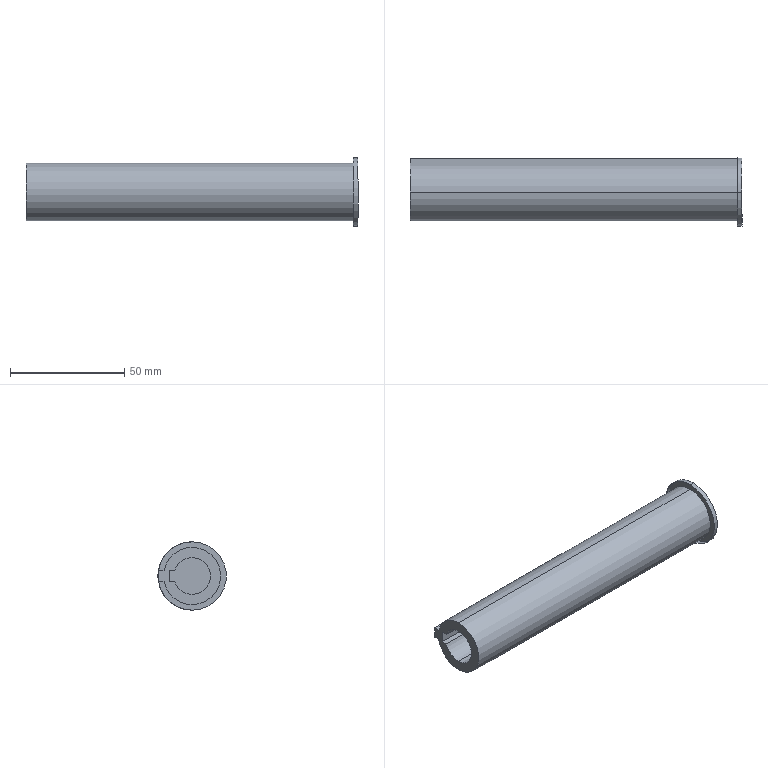Component | SolidWorks | CrushingCutterBar-1 | 1 solid | 18 faces | box 145 x 29.84 x 29.84 mm | volume 42913 mm3 | plane 10 | cylinder 8 | commonest cylinder face diameters 16 x3 25 x3 29.838 x2
STEP:
#1=CARTESIAN_POINT('',(20.913,13.193,-1.965));
#2=VERTEX_POINT('',#1);
#3=CARTESIAN_POINT('',(20.913,13.193,-0.7906));
#4=VERTEX_POINT('',#3);
#5=CARTESIAN_POINT('',(20.913,13.193,-1.378));
#6=DIRECTION('',(1.,0.,0.));
#7=DIRECTION('',(0.,0.,-1.));
#8=AXIS2_PLACEMENT_3D('',#5,#6,#7);
#9=CIRCLE('',#8,0.5874);
#10=EDGE_CURVE('',#2,#4,#9,.T.);
#11=ORIENTED_EDGE('',*,*,#10,.F.);
#12=CARTESIAN_POINT('',(20.834,13.193,-1.965));
#13=VERTEX_POINT('',#12);
#14=CARTESIAN_POINT('',(20.913,13.193,-1.965));
#15=DIRECTION('',(-1.,-0.,-0.));
#16=VECTOR('',#15,39.37);
#17=LINE('',#14,#16);
#18=EDGE_CURVE('',#2,#13,#17,.T.);
#19=ORIENTED_EDGE('',*,*,#18,.T.);
#20=CARTESIAN_POINT('',(20.834,13.772,-1.476));
#21=VERTEX_POINT('',#20);
#22=CARTESIAN_POINT('',(20.834,13.193,-1.378));
#23=DIRECTION('',(1.,0.,0.));
#24=DIRECTION('',(0.,0.,-1.));
#25=AXIS2_PLACEMENT_3D('',#22,#23,#24);
#26=CIRCLE('',#25,0.5874);
#27=EDGE_CURVE('',#13,#21,#26,.T.);
#28=ORIENTED_EDGE('',*,*,#27,.T.);
#29=CARTESIAN_POINT('',(20.834,13.193,-0.7906));
#30=VERTEX_POINT('',#29);
#31=CARTESIAN_POINT('',(20.834,13.193,-1.378));
#32=DIRECTION('',(1.,0.,0.));
#33=DIRECTION('',(0.,0.,-1.));
#34=AXIS2_PLACEMENT_3D('',#31,#32,#33);
#35=CIRCLE('',#34,0.5874);
#36=EDGE_CURVE('',#21,#30,#35,.T.);
#37=ORIENTED_EDGE('',*,*,#36,.T.);
#38=CARTESIAN_POINT('',(20.913,13.193,-0.7906));
#39=DIRECTION('',(-1.,-0.,-0.));
#40=VECTOR('',#39,39.37);
#41=LINE('',#38,#40);
#42=EDGE_CURVE('',#4,#30,#41,.T.);
#43=ORIENTED_EDGE('',*,*,#42,.F.);
#44=EDGE_LOOP('',(#11,#19,#28,#37,#43));
#45=FACE_OUTER_BOUND('',#44,.T.);
#46=CARTESIAN_POINT('',(20.913,13.193,-1.378));
#47=DIRECTION('',(-1.,-0.,-0.));
#48=DIRECTION('',(0.,0.,1.));
#49=AXIS2_PLACEMENT_3D('',#46,#47,#48);
#50=CYLINDRICAL_SURFACE('',#49,0.5874);
#51=ADVANCED_FACE('',(#45),#50,.T.);
#52=CARTESIAN_POINT('',(20.834,13.193,-1.063));
#53=VERTEX_POINT('',#52);
#54=CARTESIAN_POINT('',(20.834,13.193,-1.693));
#55=VERTEX_POINT('',#54);
#56=CARTESIAN_POINT('',(20.834,13.193,-1.378));
#57=DIRECTION('',(1.,0.,0.));
#58=DIRECTION('',(0.,0.,-1.));
#59=AXIS2_PLACEMENT_3D('',#56,#57,#58);
#60=CIRCLE('',#59,0.315);
#61=EDGE_CURVE('',#53,#55,#60,.T.);
#62=ORIENTED_EDGE('',*,*,#61,.T.);
#63=CARTESIAN_POINT('',(15.204,13.193,-1.693));
#64=VERTEX_POINT('',#63);
#65=CARTESIAN_POINT('',(20.834,13.193,-1.693));
#66=DIRECTION('',(-1.,-0.,-0.));
#67=VECTOR('',#66,39.37);
#68=LINE('',#65,#67);
#69=EDGE_CURVE('',#55,#64,#68,.T.);
#70=ORIENTED_EDGE('',*,*,#69,.T.);
#71=CARTESIAN_POINT('',(15.204,13.193,-1.063));
#72=VERTEX_POINT('',#71);
#73=CARTESIAN_POINT('',(15.204,13.193,-1.378));
#74=DIRECTION('',(1.,0.,0.));
#75=DIRECTION('',(0.,0.,-1.));
#76=AXIS2_PLACEMENT_3D('',#73,#74,#75);
#77=CIRCLE('',#76,0.315);
#78=EDGE_CURVE('',#72,#64,#77,.T.);
#79=ORIENTED_EDGE('',*,*,#78,.F.);
#80=CARTESIAN_POINT('',(20.834,13.193,-1.063));
#81=DIRECTION('',(-1.,-0.,-0.));
#82=VECTOR('',#81,39.37);
#83=LINE('',#80,#82);
#84=EDGE_CURVE('',#53,#72,#83,.T.);
#85=ORIENTED_EDGE('',*,*,#84,.F.);
#86=EDGE_LOOP('',(#62,#70,#79,#85));
#87=FACE_OUTER_BOUND('',#86,.T.);
#88=CARTESIAN_POINT('',(20.834,13.193,-1.378));
#89=DIRECTION('',(-1.,-0.,-0.));
#90=DIRECTION('',(0.,0.,1.));
#91=AXIS2_PLACEMENT_3D('',#88,#89,#90);
#92=CYLINDRICAL_SURFACE('',#91,0.315);
#93=ADVANCED_FACE('',(#87),#92,.F.);
#94=CARTESIAN_POINT('',(20.834,13.492,-1.28));
#95=VERTEX_POINT('',#94);
#96=CARTESIAN_POINT('',(20.834,13.193,-1.378));
#97=DIRECTION('',(1.,0.,0.));
#98=DIRECTION('',(0.,0.,-1.));
#99=AXIS2_PLACEMENT_3D('',#96,#97,#98);
#100=CIRCLE('',#99,0.315);
#101=EDGE_CURVE('',#95,#53,#100,.T.);
#102=ORIENTED_EDGE('',*,*,#101,.T.);
#103=ORIENTED_EDGE('',*,*,#84,.T.);
#104=CARTESIAN_POINT('',(15.204,13.492,-1.28));
#105=VERTEX_POINT('',#104);
#106=CARTESIAN_POINT('',(15.204,13.193,-1.378));
#107=DIRECTION('',(1.,0.,0.));
#108=DIRECTION('',(0.,0.,-1.));
#109=AXIS2_PLACEMENT_3D('',#106,#107,#108);
#110=CIRCLE('',#109,0.315);
#111=EDGE_CURVE('',#105,#72,#110,.T.);
#112=ORIENTED_EDGE('',*,*,#111,.F.);
#113=CARTESIAN_POINT('',(20.834,13.492,-1.28));
#114=DIRECTION('',(-1.,-0.,-0.));
#115=VECTOR('',#114,39.37);
#116=LINE('',#113,#115);
#117=EDGE_CURVE('',#95,#105,#116,.T.);
#118=ORIENTED_EDGE('',*,*,#117,.F.);
#119=EDGE_LOOP('',(#102,#103,#112,#118));
#120=FACE_OUTER_BOUND('',#119,.T.);
#121=CARTESIAN_POINT('',(20.834,13.193,-1.378));
#122=DIRECTION('',(-1.,-0.,-0.));
#123=DIRECTION('',(0.,0.,1.));
#124=AXIS2_PLACEMENT_3D('',#121,#122,#123);
#125=CYLINDRICAL_SURFACE('',#124,0.315);
#126=ADVANCED_FACE('',(#120),#125,.F.);
#127=CARTESIAN_POINT('',(20.834,13.193,-1.87));
#128=VERTEX_POINT('',#127);
#129=CARTESIAN_POINT('',(20.834,13.675,-1.476));
#130=VERTEX_POINT('',#129);
#131=CARTESIAN_POINT('',(20.834,13.193,-1.378));
#132=DIRECTION('',(1.,0.,0.));
#133=DIRECTION('',(0.,0.,-1.));
#134=AXIS2_PLACEMENT_3D('',#131,#132,#133);
#135=CIRCLE('',#134,0.4921);
#136=EDGE_CURVE('',#128,#130,#135,.T.);
#137=ORIENTED_EDGE('',*,*,#136,.F.);
#138=CARTESIAN_POINT('',(15.204,13.193,-1.87));
#139=VERTEX_POINT('',#138);
#140=CARTESIAN_POINT('',(20.834,13.193,-1.87));
#141=DIRECTION('',(-1.,-0.,-0.));
#142=VECTOR('',#141,39.37);
#143=LINE('',#140,#142);
#144=EDGE_CURVE('',#128,#139,#143,.T.);
#145=ORIENTED_EDGE('',*,*,#144,.T.);
#146=CARTESIAN_POINT('',(15.204,13.675,-1.476));
#147=VERTEX_POINT('',#146);
#148=CARTESIAN_POINT('',(15.204,13.193,-1.378));
#149=DIRECTION('',(1.,0.,0.));
#150=DIRECTION('',(0.,0.,-1.));
#151=AXIS2_PLACEMENT_3D('',#148,#149,#150);
#152=CIRCLE('',#151,0.4921);
#153=EDGE_CURVE('',#139,#147,#152,.T.);
#154=ORIENTED_EDGE('',*,*,#153,.T.);
#155=CARTESIAN_POINT('',(20.834,13.675,-1.476));
#156=DIRECTION('',(-1.,-0.,-0.));
#157=VECTOR('',#156,39.37);
#158=LINE('',#155,#157);
#159=EDGE_CURVE('',#130,#147,#158,.T.);
#160=ORIENTED_EDGE('',*,*,#159,.F.);
#161=EDGE_LOOP('',(#137,#145,#154,#160));
#162=FACE_OUTER_BOUND('',#161,.T.);
#163=CARTESIAN_POINT('',(20.834,13.193,-1.378));
#164=DIRECTION('',(-1.,-0.,-0.));
#165=DIRECTION('',(0.,0.,1.));
#166=AXIS2_PLACEMENT_3D('',#163,#164,#165);
#167=CYLINDRICAL_SURFACE('',#166,0.4921);
#168=ADVANCED_FACE('',(#162),#167,.T.);
#169=ORIENTED_EDGE('',*,*,#144,.F.);
#170=CARTESIAN_POINT('',(20.834,13.193,-0.8858));
#171=VERTEX_POINT('',#170);
#172=CARTESIAN_POINT('',(20.834,13.193,-1.378));
#173=DIRECTION('',(1.,0.,0.));
#174=DIRECTION('',(0.,0.,-1.));
#175=AXIS2_PLACEMENT_3D('',#172,#173,#174);
#176=CIRCLE('',#175,0.4921);
#177=EDGE_CURVE('',#171,#128,#176,.T.);
#178=ORIENTED_EDGE('',*,*,#177,.F.);
#179=CARTESIAN_POINT('',(15.204,13.193,-0.8858));
#180=VERTEX_POINT('',#179);
#181=CARTESIAN_POINT('',(20.834,13.193,-0.8858));
#182=DIRECTION('',(-1.,-0.,-0.));
#183=VECTOR('',#182,39.37);
#184=LINE('',#181,#183);
#185=EDGE_CURVE('',#171,#180,#184,.T.);
#186=ORIENTED_EDGE('',*,*,#185,.T.);
#187=CARTESIAN_POINT('',(15.204,13.193,-1.378));
#188=DIRECTION('',(1.,0.,0.));
#189=DIRECTION('',(0.,0.,-1.));
#190=AXIS2_PLACEMENT_3D('',#187,#188,#189);
#191=CIRCLE('',#190,0.4921);
#192=EDGE_CURVE('',#180,#139,#191,.T.);
#193=ORIENTED_EDGE('',*,*,#192,.T.);
#194=EDGE_LOOP('',(#169,#178,#186,#193));
#195=FACE_OUTER_BOUND('',#194,.T.);
#196=CARTESIAN_POINT('',(20.834,13.193,-1.378));
#197=DIRECTION('',(-1.,-0.,-0.));
#198=DIRECTION('',(0.,0.,1.));
#199=AXIS2_PLACEMENT_3D('',#196,#197,#198);
#200=CYLINDRICAL_SURFACE('',#199,0.4921);
#201=ADVANCED_FACE('',(#195),#200,.T.);
#202=CARTESIAN_POINT('',(15.204,13.675,-1.28));
#203=VERTEX_POINT('',#202);
#204=CARTESIAN_POINT('',(15.204,13.193,-1.378));
#205=DIRECTION('',(1.,0.,0.));
#206=DIRECTION('',(0.,0.,-1.));
#207=AXIS2_PLACEMENT_3D('',#204,#205,#206);
#208=CIRCLE('',#207,0.4921);
#209=EDGE_CURVE('',#203,#180,#208,.T.);
#210=ORIENTED_EDGE('',*,*,#209,.F.);
#211=CARTESIAN_POINT('',(15.204,13.772,-1.28));
#212=VERTEX_POINT('',#211);
#213=CARTESIAN_POINT('',(15.204,13.675,-1.28));
#214=DIRECTION('',(0.,-1.,-0.));
#215=VECTOR('',#214,39.37);
#216=LINE('',#213,#215);
#217=EDGE_CURVE('',#212,#203,#216,.T.);
#218=ORIENTED_EDGE('',*,*,#217,.F.);
#219=CARTESIAN_POINT('',(15.204,13.772,-1.476));
#220=VERTEX_POINT('',#219);
#221=CARTESIAN_POINT('',(15.204,13.772,-1.28));
#222=DIRECTION('',(-0.,-0.,1.));
#223=VECTOR('',#222,39.37);
#224=LINE('',#221,#223);
#225=EDGE_CURVE('',#220,#212,#224,.T.);
#226=ORIENTED_EDGE('',*,*,#225,.F.);
#227=CARTESIAN_POINT('',(15.204,13.772,-1.476));
#228=DIRECTION('',(-0.,1.,0.));
#229=VECTOR('',#228,39.37);
#230=LINE('',#227,#229);
#231=EDGE_CURVE('',#147,#220,#230,.T.);
#232=ORIENTED_EDGE('',*,*,#231,.F.);
#233=ORIENTED_EDGE('',*,*,#153,.F.);
#234=ORIENTED_EDGE('',*,*,#192,.F.);
#235=EDGE_LOOP('',(#210,#218,#226,#232,#233,#234));
#236=FACE_OUTER_BOUND('',#235,.T.);
#237=ORIENTED_EDGE('',*,*,#111,.T.);
#238=ORIENTED_EDGE('',*,*,#78,.T.);
#239=CARTESIAN_POINT('',(15.204,13.492,-1.476));
#240=VERTEX_POINT('',#239);
#241=CARTESIAN_POINT('',(15.204,13.193,-1.378));
#242=DIRECTION('',(1.,0.,0.));
#243=DIRECTION('',(0.,0.,-1.));
#244=AXIS2_PLACEMENT_3D('',#241,#242,#243);
#245=CIRCLE('',#244,0.315);
#246=EDGE_CURVE('',#64,#240,#245,.T.);
#247=ORIENTED_EDGE('',*,*,#246,.T.);
#248=CARTESIAN_POINT('',(15.204,13.589,-1.476));
#249=VERTEX_POINT('',#248);
#250=CARTESIAN_POINT('',(15.204,13.589,-1.476));
#251=DIRECTION('',(-0.,1.,0.));
#252=VECTOR('',#251,39.37);
#253=LINE('',#250,#252);
#254=EDGE_CURVE('',#240,#249,#253,.T.);
#255=ORIENTED_EDGE('',*,*,#254,.T.);
#256=CARTESIAN_POINT('',(15.204,13.589,-1.28));
#257=VERTEX_POINT('',#256);
#258=CARTESIAN_POINT('',(15.204,13.589,-1.28));
#259=DIRECTION('',(-0.,-0.,1.));
#260=VECTOR('',#259,39.37);
#261=LINE('',#258,#260);
#262=EDGE_CURVE('',#249,#257,#261,.T.);
#263=ORIENTED_EDGE('',*,*,#262,.T.);
#264=CARTESIAN_POINT('',(15.204,13.492,-1.28));
#265=DIRECTION('',(0.,-1.,-0.));
#266=VECTOR('',#265,39.37);
#267=LINE('',#264,#266);
#268=EDGE_CURVE('',#257,#105,#267,.T.);
#269=ORIENTED_EDGE('',*,*,#268,.T.);
#270=EDGE_LOOP('',(#237,#238,#247,#255,#263,#269));
#271=FACE_BOUND('',#270,.T.);
#272=CARTESIAN_POINT('',(15.204,13.193,-1.378));
#273=DIRECTION('',(1.,0.,0.));
#274=DIRECTION('',(0.,0.,-1.));
#275=AXIS2_PLACEMENT_3D('',#272,#273,#274);
#276=PLANE('',#275);
#277=ADVANCED_FACE('',(#236,#271),#276,.F.);
#278=ORIENTED_EDGE('',*,*,#185,.F.);
#279=CARTESIAN_POINT('',(20.834,13.675,-1.28));
#280=VERTEX_POINT('',#279);
#281=CARTESIAN_POINT('',(20.834,13.193,-1.378));
#282=DIRECTION('',(1.,0.,0.));
#283=DIRECTION('',(0.,0.,-1.));
#284=AXIS2_PLACEMENT_3D('',#281,#282,#283);
#285=CIRCLE('',#284,0.4921);
#286=EDGE_CURVE('',#280,#171,#285,.T.);
#287=ORIENTED_EDGE('',*,*,#286,.F.);
#288=CARTESIAN_POINT('',(20.834,13.675,-1.28));
#289=DIRECTION('',(-1.,-0.,-0.));
#290=VECTOR('',#289,39.37);
#291=LINE('',#288,#290);
#292=EDGE_CURVE('',#280,#203,#291,.T.);
#293=ORIENTED_EDGE('',*,*,#292,.T.);
#294=ORIENTED_EDGE('',*,*,#209,.T.);
#295=EDGE_LOOP('',(#278,#287,#293,#294));
#296=FACE_OUTER_BOUND('',#295,.T.);
#297=CARTESIAN_POINT('',(20.834,13.193,-1.378));
#298=DIRECTION('',(-1.,-0.,-0.));
#299=DIRECTION('',(0.,0.,1.));
#300=AXIS2_PLACEMENT_3D('',#297,#298,#299);
#301=CYLINDRICAL_SURFACE('',#300,0.4921);
#302=ADVANCED_FACE('',(#296),#301,.T.);
#303=ORIENTED_EDGE('',*,*,#231,.T.);
#304=CARTESIAN_POINT('',(20.834,13.772,-1.476));
#305=DIRECTION('',(-1.,-0.,-0.));
#306=VECTOR('',#305,39.37);
#307=LINE('',#304,#306);
#308=EDGE_CURVE('',#21,#220,#307,.T.);
#309=ORIENTED_EDGE('',*,*,#308,.F.);
#310=CARTESIAN_POINT('',(20.834,13.772,-1.476));
#311=DIRECTION('',(-0.,1.,0.));
#312=VECTOR('',#311,39.37);
#313=LINE('',#310,#312);
#314=EDGE_CURVE('',#130,#21,#313,.T.);
#315=ORIENTED_EDGE('',*,*,#314,.F.);
#316=ORIENTED_EDGE('',*,*,#159,.T.);
#317=EDGE_LOOP('',(#303,#309,#315,#316));
#318=FACE_OUTER_BOUND('',#317,.T.);
#319=CARTESIAN_POINT('',(20.834,13.772,-1.476));
#320=DIRECTION('',(-0.,-0.,1.));
#321=DIRECTION('',(0.,-1.,-0.));
#322=AXIS2_PLACEMENT_3D('',#319,#320,#321);
#323=PLANE('',#322);
#324=ADVANCED_FACE('',(#318),#323,.F.);
#325=ORIENTED_EDGE('',*,*,#225,.T.);
#326=CARTESIAN_POINT('',(20.834,13.772,-1.28));
#327=VERTEX_POINT('',#326);
#328=CARTESIAN_POINT('',(20.834,13.772,-1.28));
#329=DIRECTION('',(-1.,-0.,-0.));
#330=VECTOR('',#329,39.37);
#331=LINE('',#328,#330);
#332=EDGE_CURVE('',#327,#212,#331,.T.);
#333=ORIENTED_EDGE('',*,*,#332,.F.);
#334=CARTESIAN_POINT('',(20.834,13.772,-1.28));
#335=DIRECTION('',(-0.,-0.,1.));
#336=VECTOR('',#335,39.37);
#337=LINE('',#334,#336);
#338=EDGE_CURVE('',#21,#327,#337,.T.);
#339=ORIENTED_EDGE('',*,*,#338,.F.);
#340=ORIENTED_EDGE('',*,*,#308,.T.);
#341=EDGE_LOOP('',(#325,#333,#339,#340));
#342=FACE_OUTER_BOUND('',#341,.T.);
#343=CARTESIAN_POINT('',(20.834,13.772,-1.28));
#344=DIRECTION('',(0.,-1.,-0.));
#345=DIRECTION('',(-1.,-0.,-0.));
#346=AXIS2_PLACEMENT_3D('',#343,#344,#345);
#347=PLANE('',#346);
#348=ADVANCED_FACE('',(#342),#347,.F.);
#349=ORIENTED_EDGE('',*,*,#217,.T.);
#350=ORIENTED_EDGE('',*,*,#292,.F.);
#351=CARTESIAN_POINT('',(20.834,13.675,-1.28));
#352=DIRECTION('',(0.,-1.,-0.));
#353=VECTOR('',#352,39.37);
#354=LINE('',#351,#353);
#355=EDGE_CURVE('',#327,#280,#354,.T.);
#356=ORIENTED_EDGE('',*,*,#355,.F.);
#357=ORIENTED_EDGE('',*,*,#332,.T.);
#358=EDGE_LOOP('',(#349,#350,#356,#357));
#359=FACE_OUTER_BOUND('',#358,.T.);
#360=CARTESIAN_POINT('',(20.834,13.675,-1.28));
#361=DIRECTION('',(0.,0.,-1.));
#362=DIRECTION('',(-1.,-0.,-0.));
#363=AXIS2_PLACEMENT_3D('',#360,#361,#362);
#364=PLANE('',#363);
#365=ADVANCED_FACE('',(#359),#364,.F.);
#366=ORIENTED_EDGE('',*,*,#69,.F.);
#367=CARTESIAN_POINT('',(20.834,13.492,-1.476));
#368=VERTEX_POINT('',#367);
#369=CARTESIAN_POINT('',(20.834,13.193,-1.378));
#370=DIRECTION('',(1.,0.,0.));
#371=DIRECTION('',(0.,0.,-1.));
#372=AXIS2_PLACEMENT_3D('',#369,#370,#371);
#373=CIRCLE('',#372,0.315);
#374=EDGE_CURVE('',#55,#368,#373,.T.);
#375=ORIENTED_EDGE('',*,*,#374,.T.);
#376=CARTESIAN_POINT('',(20.834,13.492,-1.476));
#377=DIRECTION('',(-1.,-0.,-0.));
#378=VECTOR('',#377,39.37);
#379=LINE('',#376,#378);
#380=EDGE_CURVE('',#368,#240,#379,.T.);
#381=ORIENTED_EDGE('',*,*,#380,.T.);
#382=ORIENTED_EDGE('',*,*,#246,.F.);
#383=EDGE_LOOP('',(#366,#375,#381,#382));
#384=FACE_OUTER_BOUND('',#383,.T.);
#385=CARTESIAN_POINT('',(20.834,13.193,-1.378));
#386=DIRECTION('',(-1.,-0.,-0.));
#387=DIRECTION('',(0.,0.,1.));
#388=AXIS2_PLACEMENT_3D('',#385,#386,#387);
#389=CYLINDRICAL_SURFACE('',#388,0.315);
#390=ADVANCED_FACE('',(#384),#389,.F.);
#391=ORIENTED_EDGE('',*,*,#254,.F.);
#392=ORIENTED_EDGE('',*,*,#380,.F.);
#393=CARTESIAN_POINT('',(20.834,13.589,-1.476));
#394=VERTEX_POINT('',#393);
#395=CARTESIAN_POINT('',(20.834,13.589,-1.476));
#396=DIRECTION('',(-0.,1.,0.));
#397=VECTOR('',#396,39.37);
#398=LINE('',#395,#397);
#399=EDGE_CURVE('',#368,#394,#398,.T.);
#400=ORIENTED_EDGE('',*,*,#399,.T.);
#401=CARTESIAN_POINT('',(20.834,13.589,-1.476));
#402=DIRECTION('',(-1.,-0.,-0.));
#403=VECTOR('',#402,39.37);
#404=LINE('',#401,#403);
#405=EDGE_CURVE('',#394,#249,#404,.T.);
#406=ORIENTED_EDGE('',*,*,#405,.T.);
#407=EDGE_LOOP('',(#391,#392,#400,#406));
#408=FACE_OUTER_BOUND('',#407,.T.);
#409=CARTESIAN_POINT('',(20.834,13.589,-1.476));
#410=DIRECTION('',(-0.,-0.,1.));
#411=DIRECTION('',(0.,-1.,-0.));
#412=AXIS2_PLACEMENT_3D('',#409,#410,#411);
#413=PLANE('',#412);
#414=ADVANCED_FACE('',(#408),#413,.T.);
#415=ORIENTED_EDGE('',*,*,#262,.F.);
#416=ORIENTED_EDGE('',*,*,#405,.F.);
#417=CARTESIAN_POINT('',(20.834,13.589,-1.28));
#418=VERTEX_POINT('',#417);
#419=CARTESIAN_POINT('',(20.834,13.589,-1.28));
#420=DIRECTION('',(-0.,-0.,1.));
#421=VECTOR('',#420,39.37);
#422=LINE('',#419,#421);
#423=EDGE_CURVE('',#394,#418,#422,.T.);
#424=ORIENTED_EDGE('',*,*,#423,.T.);
#425=CARTESIAN_POINT('',(20.834,13.589,-1.28));
#426=DIRECTION('',(-1.,-0.,-0.));
#427=VECTOR('',#426,39.37);
#428=LINE('',#425,#427);
#429=EDGE_CURVE('',#418,#257,#428,.T.);
#430=ORIENTED_EDGE('',*,*,#429,.T.);
#431=EDGE_LOOP('',(#415,#416,#424,#430));
#432=FACE_OUTER_BOUND('',#431,.T.);
#433=CARTESIAN_POINT('',(20.834,13.589,-1.28));
#434=DIRECTION('',(0.,-1.,-0.));
#435=DIRECTION('',(-1.,-0.,-0.));
#436=AXIS2_PLACEMENT_3D('',#433,#434,#435);
#437=PLANE('',#436);
#438=ADVANCED_FACE('',(#432),#437,.T.);
#439=ORIENTED_EDGE('',*,*,#268,.F.);
#440=ORIENTED_EDGE('',*,*,#429,.F.);
#441=CARTESIAN_POINT('',(20.834,13.492,-1.28));
#442=DIRECTION('',(0.,-1.,-0.));
#443=VECTOR('',#442,39.37);
#444=LINE('',#441,#443);
#445=EDGE_CURVE('',#418,#95,#444,.T.);
#446=ORIENTED_EDGE('',*,*,#445,.T.);
#447=ORIENTED_EDGE('',*,*,#117,.T.);
#448=EDGE_LOOP('',(#439,#440,#446,#447));
#449=FACE_OUTER_BOUND('',#448,.T.);
#450=CARTESIAN_POINT('',(20.834,13.492,-1.28));
#451=DIRECTION('',(0.,0.,-1.));
#452=DIRECTION('',(-1.,-0.,-0.));
#453=AXIS2_PLACEMENT_3D('',#450,#451,#452);
#454=PLANE('',#453);
#455=ADVANCED_FACE('',(#449),#454,.T.);
#456=ORIENTED_EDGE('',*,*,#399,.F.);
#457=ORIENTED_EDGE('',*,*,#374,.F.);
#458=ORIENTED_EDGE('',*,*,#61,.F.);
#459=ORIENTED_EDGE('',*,*,#101,.F.);
#460=ORIENTED_EDGE('',*,*,#445,.F.);
#461=ORIENTED_EDGE('',*,*,#423,.F.);
#462=EDGE_LOOP('',(#456,#457,#458,#459,#460,#461));
#463=FACE_OUTER_BOUND('',#462,.T.);
#464=CARTESIAN_POINT('',(20.834,13.193,-1.378));
#465=DIRECTION('',(1.,0.,0.));
#466=DIRECTION('',(0.,0.,-1.));
#467=AXIS2_PLACEMENT_3D('',#464,#465,#466);
#468=PLANE('',#467);
#469=ADVANCED_FACE('',(#463),#468,.F.);
#470=ORIENTED_EDGE('',*,*,#18,.F.);
#471=CARTESIAN_POINT('',(20.913,13.193,-1.378));
#472=DIRECTION('',(1.,0.,0.));
#473=DIRECTION('',(0.,0.,-1.));
#474=AXIS2_PLACEMENT_3D('',#471,#472,#473);
#475=CIRCLE('',#474,0.5874);
#476=EDGE_CURVE('',#4,#2,#475,.T.);
#477=ORIENTED_EDGE('',*,*,#476,.F.);
#478=ORIENTED_EDGE('',*,*,#42,.T.);
#479=CARTESIAN_POINT('',(20.834,13.193,-1.378));
#480=DIRECTION('',(1.,0.,0.));
#481=DIRECTION('',(0.,0.,-1.));
#482=AXIS2_PLACEMENT_3D('',#479,#480,#481);
#483=CIRCLE('',#482,0.5874);
#484=EDGE_CURVE('',#30,#13,#483,.T.);
#485=ORIENTED_EDGE('',*,*,#484,.T.);
#486=EDGE_LOOP('',(#470,#477,#478,#485));
#487=FACE_OUTER_BOUND('',#486,.T.);
#488=CARTESIAN_POINT('',(20.913,13.193,-1.378));
#489=DIRECTION('',(-1.,-0.,-0.));
#490=DIRECTION('',(0.,0.,1.));
#491=AXIS2_PLACEMENT_3D('',#488,#489,#490);
#492=CYLINDRICAL_SURFACE('',#491,0.5874);
#493=ADVANCED_FACE('',(#487),#492,.T.);
#494=ORIENTED_EDGE('',*,*,#476,.T.);
#495=ORIENTED_EDGE('',*,*,#10,.T.);
#496=EDGE_LOOP('',(#494,#495));
#497=FACE_OUTER_BOUND('',#496,.T.);
#498=CARTESIAN_POINT('',(20.913,13.193,-1.378));
#499=DIRECTION('',(1.,0.,0.));
#500=DIRECTION('',(0.,0.,-1.));
#501=AXIS2_PLACEMENT_3D('',#498,#499,#500);
#502=PLANE('',#501);
#503=ADVANCED_FACE('',(#497),#502,.T.);
#504=ORIENTED_EDGE('',*,*,#355,.T.);
#505=ORIENTED_EDGE('',*,*,#286,.T.);
#506=ORIENTED_EDGE('',*,*,#177,.T.);
#507=ORIENTED_EDGE('',*,*,#136,.T.);
#508=ORIENTED_EDGE('',*,*,#314,.T.);
#509=ORIENTED_EDGE('',*,*,#27,.F.);
#510=ORIENTED_EDGE('',*,*,#484,.F.);
#511=ORIENTED_EDGE('',*,*,#36,.F.);
#512=ORIENTED_EDGE('',*,*,#338,.T.);
#513=EDGE_LOOP('',(#504,#505,#506,#507,#508,#509,#510,#511,#512));
#514=FACE_OUTER_BOUND('',#513,.T.);
#515=CARTESIAN_POINT('',(20.834,13.193,-1.378));
#516=DIRECTION('',(1.,0.,0.));
#517=DIRECTION('',(0.,0.,-1.));
#518=AXIS2_PLACEMENT_3D('',#515,#516,#517);
#519=PLANE('',#518);
#520=ADVANCED_FACE('',(#514),#519,.F.);
#521=CLOSED_SHELL('',(#51,#93,#126,#168,#201,#277,#302,#324,#348,#365,#390,#414,#438,#455,#469,#493,#503,#520));
#522=MANIFOLD_SOLID_BREP('',#521);
#523=CARTESIAN_POINT('',(0.,0.,0.));
#524=DIRECTION('',(0.,0.,1.));
#525=DIRECTION('',(1.,0.,0.));
#526=AXIS2_PLACEMENT_3D('',#523,#524,#525);
#527=(LENGTH_UNIT()NAMED_UNIT(*)SI_UNIT($,.METRE.));
#528=LENGTH_MEASURE_WITH_UNIT(LENGTH_MEASURE(0.0254),#527);
#529=DIMENSIONAL_EXPONENTS(1.,0.,0.,0.,0.,0.,0.);
#530=(CONVERSION_BASED_UNIT('',#528)LENGTH_UNIT()NAMED_UNIT(#529));
#531=UNCERTAINTY_MEASURE_WITH_UNIT(LENGTH_MEASURE(0.00001),#530,'','');
#532=(NAMED_UNIT(*)PLANE_ANGLE_UNIT()SI_UNIT($,.RADIAN.));
#533=(NAMED_UNIT(*)SI_UNIT($,.STERADIAN.)SOLID_ANGLE_UNIT());
#534=(GEOMETRIC_REPRESENTATION_CONTEXT(3)GLOBAL_UNCERTAINTY_ASSIGNED_CONTEXT((#531))GLOBAL_UNIT_ASSIGNED_CONTEXT((#530,#532,#533))REPRESENTATION_CONTEXT('',''));
#535=ADVANCED_BREP_SHAPE_REPRESENTATION('',(#522,#526),#534);
#536=COLOUR_RGB('',0.7922,0.8196,0.9333);
#537=FILL_AREA_STYLE_COLOUR('',#536);
#538=FILL_AREA_STYLE('',(#537));
#539=SURFACE_STYLE_FILL_AREA(#538);
#540=SURFACE_SIDE_STYLE('',(#539));
#541=SURFACE_STYLE_USAGE(.BOTH.,#540);
#542=PRESENTATION_STYLE_ASSIGNMENT((#541));
#543=STYLED_ITEM('',(#542),#522);
#544=(LENGTH_UNIT()NAMED_UNIT(*)SI_UNIT($,.METRE.));
#545=LENGTH_MEASURE_WITH_UNIT(LENGTH_MEASURE(0.0254),#544);
#546=DIMENSIONAL_EXPONENTS(1.,0.,0.,0.,0.,0.,0.);
#547=(CONVERSION_BASED_UNIT('',#545)LENGTH_UNIT()NAMED_UNIT(#546));
#548=UNCERTAINTY_MEASURE_WITH_UNIT(LENGTH_MEASURE(0.00001),#547,'','');
#549=(NAMED_UNIT(*)PLANE_ANGLE_UNIT()SI_UNIT($,.RADIAN.));
#550=(NAMED_UNIT(*)SI_UNIT($,.STERADIAN.)SOLID_ANGLE_UNIT());
#551=(GEOMETRIC_REPRESENTATION_CONTEXT(3)GLOBAL_UNCERTAINTY_ASSIGNED_CONTEXT((#548))GLOBAL_UNIT_ASSIGNED_CONTEXT((#547,#549,#550))REPRESENTATION_CONTEXT('',''));
#552=MECHANICAL_DESIGN_GEOMETRIC_PRESENTATION_REPRESENTATION('',(#543),#551);
#553=PRESENTATION_LAYER_ASSIGNMENT('','',(#543));